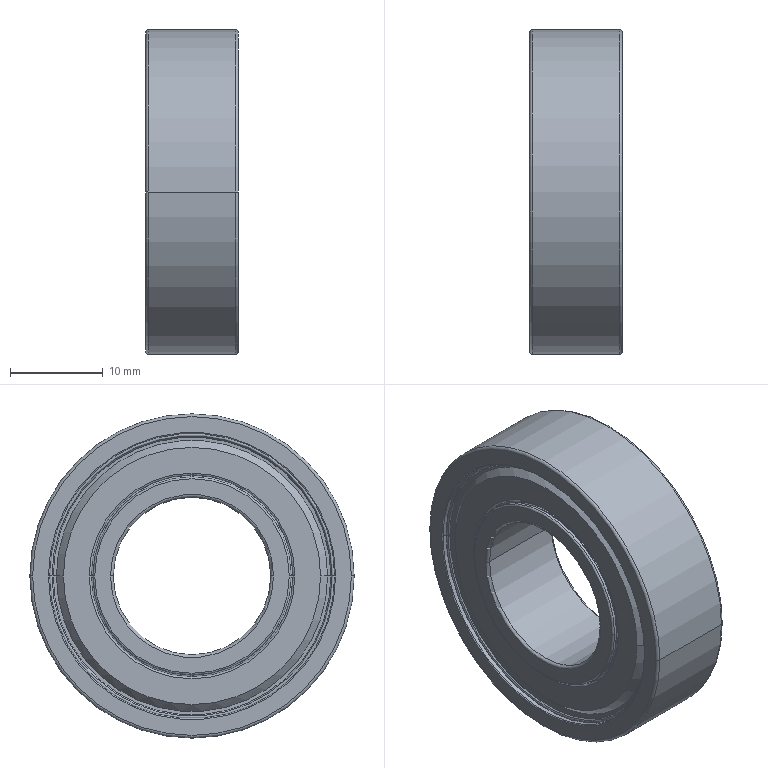Component | SolidWorks | CCD11-00TensioningAssembly-1_CCD6003ZZ-1 | 1 solid | 80 faces | box 10 x 35 x 35 mm | volume 5935 mm3 | torus 30 | cylinder 22 | cone 20 | plane 8 | commonest cylinder face diameters 29.4 x4 22.6 x4 22.2 x2 21.8 x2 30.8 x2 35 x2 17 x2 21.4 x2
build123d program:
from build123d import *


with BuildPart() as part:
    # Sketch1 → Revolve1 (revolve)
    with BuildSketch(Plane.XY, mode=Mode.PRIVATE) as revolve1_sk:
        with BuildLine():
            Line((1.503, 14.7), (2.803, 14.7))
            ThreePointArc((2.803, 14.7), (2.222, 13), (2.803, 11.3))
            Line((2.803, 11.3), (1.638, 11.3))
            ThreePointArc((1.638, 11.3), (1.523, 11.264), (1.45, 11.168))
            Line((1.45, 11.168), (1.182, 10.432))
            ThreePointArc((1.182, 10.432), (1.109, 10.336), (0.9939, 10.3))
            Line((0.9939, 10.3), (0.9288, 10.3))
            ThreePointArc((0.9288, 10.3), (0.8443, 10.319), (0.7756, 10.371))
            Line((0.7756, 10.371), (0.5, 10.7))
            Line((0.5, 10.7), (0.2, 10.7))
            ThreePointArc((0.2, 10.7), (0.05858, 10.641), (0, 10.5))
            Line((0, 10.5), (0, 8.8))
            ThreePointArc((0, 8.8), (0.08787, 8.588), (0.3, 8.5))
            Line((0.3, 8.5), (9.7, 8.5))
            ThreePointArc((9.7, 8.5), (9.912, 8.588), (10, 8.8))
            Line((10, 8.8), (10, 11.3))
            Line((10, 11.3), (7.197, 11.3))
            ThreePointArc((7.197, 11.3), (7.778, 13), (7.197, 14.7))
            Line((7.197, 14.7), (10, 14.7))
            Line((10, 14.7), (10, 17.2))
            ThreePointArc((10, 17.2), (9.912, 17.412), (9.7, 17.5))
            Line((9.7, 17.5), (0.3, 17.5))
            ThreePointArc((0.3, 17.5), (0.08787, 17.412), (0, 17.2))
            Line((0, 17.2), (0, 15.5))
            ThreePointArc((0, 15.5), (0.02929, 15.429), (0.1, 15.4))
            Line((0.1, 15.4), (0.56, 15.4))
            ThreePointArc((0.56, 15.4), (0.514, 15.254), (0.5849, 15.118))
            Line((0.5849, 15.118), (0.738, 14.99))
            Line((0.738, 14.99), (0.866, 15.143))
            Line((0.866, 15.143), (0.713, 15.271))
            Line((0.713, 15.271), (0.9634, 15.569))
            ThreePointArc((0.9634, 15.569), (1.072, 15.6), (1.14, 15.51))
            Line((1.14, 15.51), (1.183, 14.633))
            Line((1.183, 14.633), (0.4329, 13.883))
            Line((0.4329, 13.883), (0.4329, 11.1))
            ThreePointArc((0.4329, 11.1), (0.4915, 10.959), (0.6329, 10.9))
            Line((0.6329, 10.9), (1.083, 10.9))
            Line((1.083, 10.9), (1.083, 11.1))
            Line((1.083, 11.1), (0.633, 11.1))
            Line((0.633, 11.1), (0.633, 13.8))
            Line((0.633, 13.8), (1.383, 14.55))
            Line((1.383, 14.55), (1.383, 15.02))
            Line((1.383, 15.02), (1.403, 14.791))
            ThreePointArc((1.403, 14.791), (1.435, 14.726), (1.503, 14.7))
        make_face()
    revolve(revolve1_sk.sketch.rotate(Axis((-0.00125, 0, 0), (1, 0, 0)), 270), axis=Axis((-0.00125, 0, 0), (1, 0, 0)))


solid = part.part

# Placed as in the assembly
solid = solid.moved(Location((-354.121, 107.251, 149), (0, 0, 0)))